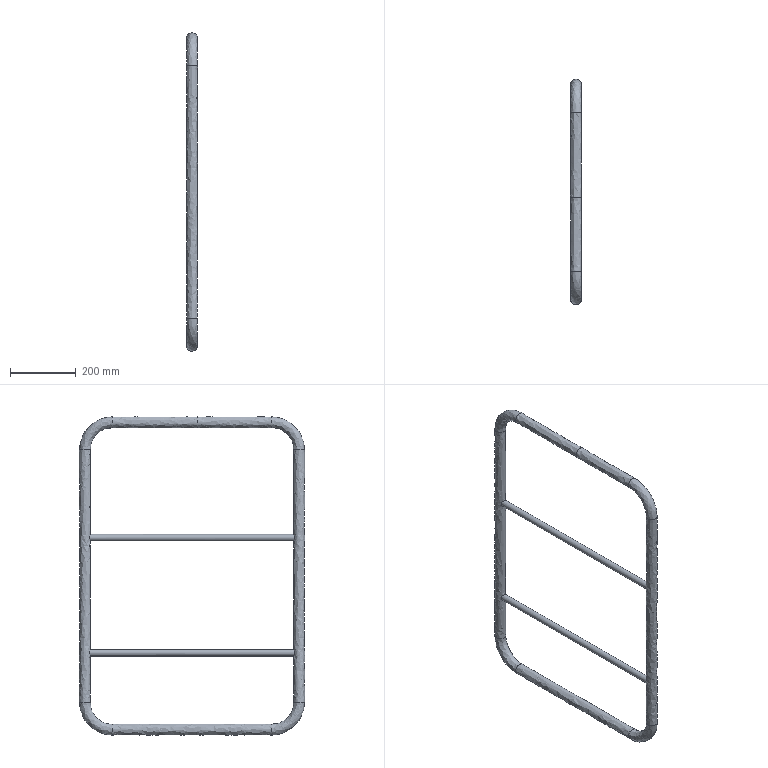Component | NX | 43_6_1_2 | 1 solid | 11 faces | volume 3515577 mm3 | spline 9 | cylinder 2 | commonest cylinder face diameters 20 x2